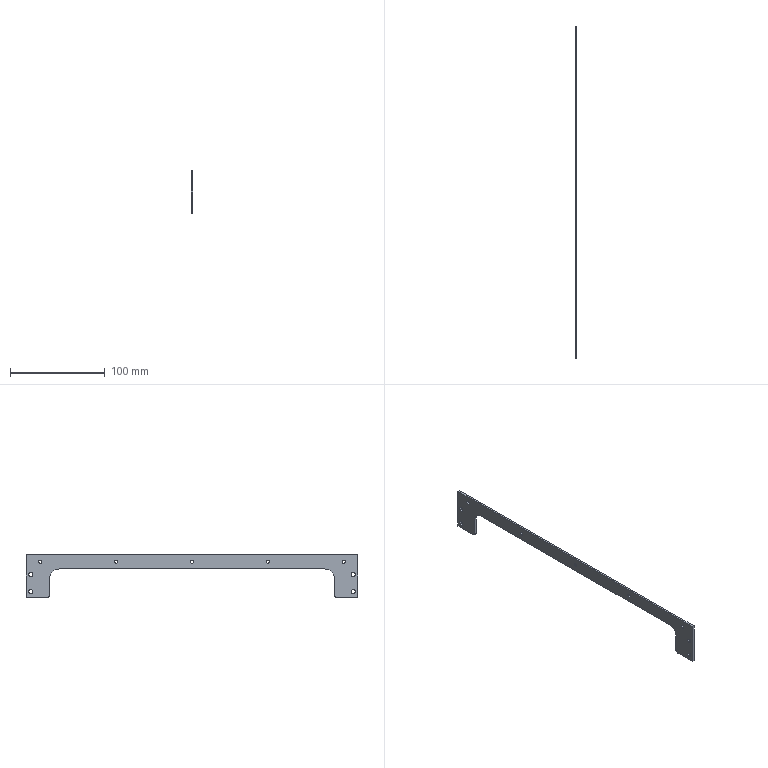Component | SolidWorks | AUTO-SpinDryWashing-01-03000009-1 | 1 solid | 32 faces | box 2 x 350 x 45 mm | volume 13360 mm3 | cylinder 22 | plane 10 | commonest cylinder face diameters 3.4 x10 4.5 x8 20 x2 6 x2 | material AISI 304
build123d program:
from build123d import *

# Parameters (mm, degrees)
SKETCH1_W                = 45
SKETCH1_H                = 350
BOSS_EXTRUDE1_DEPTH      = 1
M3_CLEARANCE_HOLE1_D     = 3.4
M3_CLEARANCE_HOLE1_DEPTH = 10
M3_CLEARANCE_HOLE1_TIP   = 1.021
M4_CLEARANCE_HOLE1_D     = 4.5
M4_CLEARANCE_HOLE1_DEPTH = 10
M4_CLEARANCE_HOLE1_TIP   = 1.352
SKETCH7_W                = 79.155
SKETCH7_H                = 300
CUT_EXTRUDE1_DEPTH       = 10
FILLET1_R                = 10
FILLET2_R                = 3


with BuildPart() as part:
    # Sketch1 → Boss-Extrude1 (new, symmetric)
    with BuildSketch(Plane.XY):
        Rectangle(SKETCH1_W, SKETCH1_H)
    extrude(amount=BOSS_EXTRUDE1_DEPTH, both=True)

    # M3 Clearance Hole1
    with Locations(Plane.XY.offset(1)):
        with Locations((-15, 160), (-15, 80), (-15, 0), (-15, -80), (-15, -160)):
            Hole(M3_CLEARANCE_HOLE1_D / 2, depth=M3_CLEARANCE_HOLE1_DEPTH)
            with Locations((0, 0, -(M3_CLEARANCE_HOLE1_DEPTH + M3_CLEARANCE_HOLE1_TIP / 2))):  # 118° drill point
                Cone(0, M3_CLEARANCE_HOLE1_D / 2, M3_CLEARANCE_HOLE1_TIP, mode=Mode.SUBTRACT)

    # M4 Clearance Hole1
    with Locations(Plane.XY.offset(1)):
        with Locations((-1.5, 170), (16.5, 170), (-1.5, -170), (16.5, -170)):
            Hole(M4_CLEARANCE_HOLE1_D / 2, depth=M4_CLEARANCE_HOLE1_DEPTH)
            with Locations((0, 0, -(M4_CLEARANCE_HOLE1_DEPTH + M4_CLEARANCE_HOLE1_TIP / 2))):  # 118° drill point
                Cone(0, M4_CLEARANCE_HOLE1_D / 2, M4_CLEARANCE_HOLE1_TIP, mode=Mode.SUBTRACT)

    # Sketch7 → Cut-Extrude1 (cut)
    with BuildSketch(Plane.XY.offset(1)):
        with Locations((32.077, 0)):
            Rectangle(SKETCH7_W, SKETCH7_H)
    extrude(amount=-CUT_EXTRUDE1_DEPTH, mode=Mode.SUBTRACT)

    # Fillet1
    fillet1_edges = [part.edges().sort_by_distance(p)[0] for p in [
        (-7.5, -150, 0),
        (-7.5, 150, 0),
    ]]
    fillet(fillet1_edges, radius=FILLET1_R)

    # Fillet2
    fillet2_edges = [part.edges().sort_by_distance(p)[0] for p in [
        (22.5, 150, 0),
        (22.5, -150, 0),
    ]]
    fillet(fillet2_edges, radius=FILLET2_R)


solid = part.part

# Placed as in the assembly
solid = solid.moved(Location((366, 643, 42.5), (0, 90, 0)))
STEP:
#1=CARTESIAN_POINT('',(14.37,32.008,1.821));
#2=VERTEX_POINT('',#1);
#3=CARTESIAN_POINT('',(14.37,32.008,1.644));
#4=VERTEX_POINT('',#3);
#5=CARTESIAN_POINT('',(14.37,32.008,1.732));
#6=DIRECTION('',(1.,-0.,0.));
#7=DIRECTION('',(0.,0.,-1.));
#8=AXIS2_PLACEMENT_3D('',#5,#6,#7);
#9=CIRCLE('',#8,0.08858);
#10=EDGE_CURVE('',#2,#4,#9,.T.);
#11=ORIENTED_EDGE('',*,*,#10,.F.);
#12=CARTESIAN_POINT('',(14.449,32.008,1.821));
#13=VERTEX_POINT('',#12);
#14=CARTESIAN_POINT('',(14.449,32.008,1.821));
#15=DIRECTION('',(1.,-0.,0.));
#16=VECTOR('',#15,39.37);
#17=LINE('',#14,#16);
#18=EDGE_CURVE('',#2,#13,#17,.T.);
#19=ORIENTED_EDGE('',*,*,#18,.T.);
#20=CARTESIAN_POINT('',(14.449,32.008,1.644));
#21=VERTEX_POINT('',#20);
#22=CARTESIAN_POINT('',(14.449,32.008,1.732));
#23=DIRECTION('',(1.,-0.,0.));
#24=DIRECTION('',(0.,0.,-1.));
#25=AXIS2_PLACEMENT_3D('',#22,#23,#24);
#26=CIRCLE('',#25,0.08858);
#27=EDGE_CURVE('',#13,#21,#26,.T.);
#28=ORIENTED_EDGE('',*,*,#27,.T.);
#29=CARTESIAN_POINT('',(14.449,32.008,1.644));
#30=DIRECTION('',(1.,-0.,0.));
#31=VECTOR('',#30,39.37);
#32=LINE('',#29,#31);
#33=EDGE_CURVE('',#4,#21,#32,.T.);
#34=ORIENTED_EDGE('',*,*,#33,.F.);
#35=EDGE_LOOP('',(#11,#19,#28,#34));
#36=FACE_OUTER_BOUND('',#35,.T.);
#37=CARTESIAN_POINT('',(14.449,32.008,1.732));
#38=DIRECTION('',(1.,-0.,0.));
#39=DIRECTION('',(0.,0.,-1.));
#40=AXIS2_PLACEMENT_3D('',#37,#38,#39);
#41=CYLINDRICAL_SURFACE('',#40,0.08858);
#42=ADVANCED_FACE('',(#36),#41,.F.);
#43=CARTESIAN_POINT('',(14.37,32.008,1.112));
#44=VERTEX_POINT('',#43);
#45=CARTESIAN_POINT('',(14.37,32.008,0.935));
#46=VERTEX_POINT('',#45);
#47=CARTESIAN_POINT('',(14.37,32.008,1.024));
#48=DIRECTION('',(1.,-0.,0.));
#49=DIRECTION('',(0.,0.,-1.));
#50=AXIS2_PLACEMENT_3D('',#47,#48,#49);
#51=CIRCLE('',#50,0.08858);
#52=EDGE_CURVE('',#44,#46,#51,.T.);
#53=ORIENTED_EDGE('',*,*,#52,.F.);
#54=CARTESIAN_POINT('',(14.449,32.008,1.112));
#55=VERTEX_POINT('',#54);
#56=CARTESIAN_POINT('',(14.449,32.008,1.112));
#57=DIRECTION('',(1.,-0.,0.));
#58=VECTOR('',#57,39.37);
#59=LINE('',#56,#58);
#60=EDGE_CURVE('',#44,#55,#59,.T.);
#61=ORIENTED_EDGE('',*,*,#60,.T.);
#62=CARTESIAN_POINT('',(14.449,32.008,0.935));
#63=VERTEX_POINT('',#62);
#64=CARTESIAN_POINT('',(14.449,32.008,1.024));
#65=DIRECTION('',(1.,-0.,0.));
#66=DIRECTION('',(0.,0.,-1.));
#67=AXIS2_PLACEMENT_3D('',#64,#65,#66);
#68=CIRCLE('',#67,0.08858);
#69=EDGE_CURVE('',#55,#63,#68,.T.);
#70=ORIENTED_EDGE('',*,*,#69,.T.);
#71=CARTESIAN_POINT('',(14.449,32.008,0.935));
#72=DIRECTION('',(1.,-0.,0.));
#73=VECTOR('',#72,39.37);
#74=LINE('',#71,#73);
#75=EDGE_CURVE('',#46,#63,#74,.T.);
#76=ORIENTED_EDGE('',*,*,#75,.F.);
#77=EDGE_LOOP('',(#53,#61,#70,#76));
#78=FACE_OUTER_BOUND('',#77,.T.);
#79=CARTESIAN_POINT('',(14.449,32.008,1.024));
#80=DIRECTION('',(1.,-0.,0.));
#81=DIRECTION('',(0.,0.,-1.));
#82=AXIS2_PLACEMENT_3D('',#79,#80,#81);
#83=CYLINDRICAL_SURFACE('',#82,0.08858);
#84=ADVANCED_FACE('',(#78),#83,.F.);
#85=CARTESIAN_POINT('',(14.37,18.622,1.821));
#86=VERTEX_POINT('',#85);
#87=CARTESIAN_POINT('',(14.37,18.622,1.644));
#88=VERTEX_POINT('',#87);
#89=CARTESIAN_POINT('',(14.37,18.622,1.732));
#90=DIRECTION('',(1.,-0.,0.));
#91=DIRECTION('',(0.,0.,-1.));
#92=AXIS2_PLACEMENT_3D('',#89,#90,#91);
#93=CIRCLE('',#92,0.08858);
#94=EDGE_CURVE('',#86,#88,#93,.T.);
#95=ORIENTED_EDGE('',*,*,#94,.F.);
#96=CARTESIAN_POINT('',(14.449,18.622,1.821));
#97=VERTEX_POINT('',#96);
#98=CARTESIAN_POINT('',(14.449,18.622,1.821));
#99=DIRECTION('',(1.,-0.,0.));
#100=VECTOR('',#99,39.37);
#101=LINE('',#98,#100);
#102=EDGE_CURVE('',#86,#97,#101,.T.);
#103=ORIENTED_EDGE('',*,*,#102,.T.);
#104=CARTESIAN_POINT('',(14.449,18.622,1.644));
#105=VERTEX_POINT('',#104);
#106=CARTESIAN_POINT('',(14.449,18.622,1.732));
#107=DIRECTION('',(1.,-0.,0.));
#108=DIRECTION('',(0.,0.,-1.));
#109=AXIS2_PLACEMENT_3D('',#106,#107,#108);
#110=CIRCLE('',#109,0.08858);
#111=EDGE_CURVE('',#97,#105,#110,.T.);
#112=ORIENTED_EDGE('',*,*,#111,.T.);
#113=CARTESIAN_POINT('',(14.449,18.622,1.644));
#114=DIRECTION('',(1.,-0.,0.));
#115=VECTOR('',#114,39.37);
#116=LINE('',#113,#115);
#117=EDGE_CURVE('',#88,#105,#116,.T.);
#118=ORIENTED_EDGE('',*,*,#117,.F.);
#119=EDGE_LOOP('',(#95,#103,#112,#118));
#120=FACE_OUTER_BOUND('',#119,.T.);
#121=CARTESIAN_POINT('',(14.449,18.622,1.732));
#122=DIRECTION('',(1.,-0.,0.));
#123=DIRECTION('',(0.,0.,-1.));
#124=AXIS2_PLACEMENT_3D('',#121,#122,#123);
#125=CYLINDRICAL_SURFACE('',#124,0.08858);
#126=ADVANCED_FACE('',(#120),#125,.F.);
#127=CARTESIAN_POINT('',(14.37,18.622,1.112));
#128=VERTEX_POINT('',#127);
#129=CARTESIAN_POINT('',(14.37,18.622,0.935));
#130=VERTEX_POINT('',#129);
#131=CARTESIAN_POINT('',(14.37,18.622,1.024));
#132=DIRECTION('',(1.,-0.,0.));
#133=DIRECTION('',(0.,0.,-1.));
#134=AXIS2_PLACEMENT_3D('',#131,#132,#133);
#135=CIRCLE('',#134,0.08858);
#136=EDGE_CURVE('',#128,#130,#135,.T.);
#137=ORIENTED_EDGE('',*,*,#136,.F.);
#138=CARTESIAN_POINT('',(14.449,18.622,1.112));
#139=VERTEX_POINT('',#138);
#140=CARTESIAN_POINT('',(14.449,18.622,1.112));
#141=DIRECTION('',(1.,-0.,0.));
#142=VECTOR('',#141,39.37);
#143=LINE('',#140,#142);
#144=EDGE_CURVE('',#128,#139,#143,.T.);
#145=ORIENTED_EDGE('',*,*,#144,.T.);
#146=CARTESIAN_POINT('',(14.449,18.622,0.935));
#147=VERTEX_POINT('',#146);
#148=CARTESIAN_POINT('',(14.449,18.622,1.024));
#149=DIRECTION('',(1.,-0.,0.));
#150=DIRECTION('',(0.,0.,-1.));
#151=AXIS2_PLACEMENT_3D('',#148,#149,#150);
#152=CIRCLE('',#151,0.08858);
#153=EDGE_CURVE('',#139,#147,#152,.T.);
#154=ORIENTED_EDGE('',*,*,#153,.T.);
#155=CARTESIAN_POINT('',(14.449,18.622,0.935));
#156=DIRECTION('',(1.,-0.,0.));
#157=VECTOR('',#156,39.37);
#158=LINE('',#155,#157);
#159=EDGE_CURVE('',#130,#147,#158,.T.);
#160=ORIENTED_EDGE('',*,*,#159,.F.);
#161=EDGE_LOOP('',(#137,#145,#154,#160));
#162=FACE_OUTER_BOUND('',#161,.T.);
#163=CARTESIAN_POINT('',(14.449,18.622,1.024));
#164=DIRECTION('',(1.,-0.,0.));
#165=DIRECTION('',(0.,0.,-1.));
#166=AXIS2_PLACEMENT_3D('',#163,#164,#165);
#167=CYLINDRICAL_SURFACE('',#166,0.08858);
#168=ADVANCED_FACE('',(#162),#167,.F.);
#169=CARTESIAN_POINT('',(14.37,31.614,2.331));
#170=VERTEX_POINT('',#169);
#171=CARTESIAN_POINT('',(14.37,31.614,2.197));
#172=VERTEX_POINT('',#171);
#173=CARTESIAN_POINT('',(14.37,31.614,2.264));
#174=DIRECTION('',(1.,-0.,0.));
#175=DIRECTION('',(0.,0.,-1.));
#176=AXIS2_PLACEMENT_3D('',#173,#174,#175);
#177=CIRCLE('',#176,0.06693);
#178=EDGE_CURVE('',#170,#172,#177,.T.);
#179=ORIENTED_EDGE('',*,*,#178,.F.);
#180=CARTESIAN_POINT('',(14.449,31.614,2.331));
#181=VERTEX_POINT('',#180);
#182=CARTESIAN_POINT('',(14.449,31.614,2.331));
#183=DIRECTION('',(1.,-0.,0.));
#184=VECTOR('',#183,39.37);
#185=LINE('',#182,#184);
#186=EDGE_CURVE('',#170,#181,#185,.T.);
#187=ORIENTED_EDGE('',*,*,#186,.T.);
#188=CARTESIAN_POINT('',(14.449,31.614,2.197));
#189=VERTEX_POINT('',#188);
#190=CARTESIAN_POINT('',(14.449,31.614,2.264));
#191=DIRECTION('',(1.,-0.,0.));
#192=DIRECTION('',(0.,0.,-1.));
#193=AXIS2_PLACEMENT_3D('',#190,#191,#192);
#194=CIRCLE('',#193,0.06693);
#195=EDGE_CURVE('',#181,#189,#194,.T.);
#196=ORIENTED_EDGE('',*,*,#195,.T.);
#197=CARTESIAN_POINT('',(14.449,31.614,2.197));
#198=DIRECTION('',(1.,-0.,0.));
#199=VECTOR('',#198,39.37);
#200=LINE('',#197,#199);
#201=EDGE_CURVE('',#172,#189,#200,.T.);
#202=ORIENTED_EDGE('',*,*,#201,.F.);
#203=EDGE_LOOP('',(#179,#187,#196,#202));
#204=FACE_OUTER_BOUND('',#203,.T.);
#205=CARTESIAN_POINT('',(14.449,31.614,2.264));
#206=DIRECTION('',(1.,-0.,0.));
#207=DIRECTION('',(0.,0.,-1.));
#208=AXIS2_PLACEMENT_3D('',#205,#206,#207);
#209=CYLINDRICAL_SURFACE('',#208,0.06693);
#210=ADVANCED_FACE('',(#204),#209,.F.);
#211=CARTESIAN_POINT('',(14.37,28.465,2.331));
#212=VERTEX_POINT('',#211);
#213=CARTESIAN_POINT('',(14.37,28.465,2.197));
#214=VERTEX_POINT('',#213);
#215=CARTESIAN_POINT('',(14.37,28.465,2.264));
#216=DIRECTION('',(1.,-0.,0.));
#217=DIRECTION('',(0.,0.,-1.));
#218=AXIS2_PLACEMENT_3D('',#215,#216,#217);
#219=CIRCLE('',#218,0.06693);
#220=EDGE_CURVE('',#212,#214,#219,.T.);
#221=ORIENTED_EDGE('',*,*,#220,.F.);
#222=CARTESIAN_POINT('',(14.449,28.465,2.331));
#223=VERTEX_POINT('',#222);
#224=CARTESIAN_POINT('',(14.449,28.465,2.331));
#225=DIRECTION('',(1.,-0.,0.));
#226=VECTOR('',#225,39.37);
#227=LINE('',#224,#226);
#228=EDGE_CURVE('',#212,#223,#227,.T.);
#229=ORIENTED_EDGE('',*,*,#228,.T.);
#230=CARTESIAN_POINT('',(14.449,28.465,2.197));
#231=VERTEX_POINT('',#230);
#232=CARTESIAN_POINT('',(14.449,28.465,2.264));
#233=DIRECTION('',(1.,-0.,0.));
#234=DIRECTION('',(0.,0.,-1.));
#235=AXIS2_PLACEMENT_3D('',#232,#233,#234);
#236=CIRCLE('',#235,0.06693);
#237=EDGE_CURVE('',#223,#231,#236,.T.);
#238=ORIENTED_EDGE('',*,*,#237,.T.);
#239=CARTESIAN_POINT('',(14.449,28.465,2.197));
#240=DIRECTION('',(1.,-0.,0.));
#241=VECTOR('',#240,39.37);
#242=LINE('',#239,#241);
#243=EDGE_CURVE('',#214,#231,#242,.T.);
#244=ORIENTED_EDGE('',*,*,#243,.F.);
#245=EDGE_LOOP('',(#221,#229,#238,#244));
#246=FACE_OUTER_BOUND('',#245,.T.);
#247=CARTESIAN_POINT('',(14.449,28.465,2.264));
#248=DIRECTION('',(1.,-0.,0.));
#249=DIRECTION('',(0.,0.,-1.));
#250=AXIS2_PLACEMENT_3D('',#247,#248,#249);
#251=CYLINDRICAL_SURFACE('',#250,0.06693);
#252=ADVANCED_FACE('',(#246),#251,.F.);
#253=CARTESIAN_POINT('',(14.37,25.315,2.331));
#254=VERTEX_POINT('',#253);
#255=CARTESIAN_POINT('',(14.37,25.315,2.197));
#256=VERTEX_POINT('',#255);
#257=CARTESIAN_POINT('',(14.37,25.315,2.264));
#258=DIRECTION('',(1.,-0.,0.));
#259=DIRECTION('',(0.,0.,-1.));
#260=AXIS2_PLACEMENT_3D('',#257,#258,#259);
#261=CIRCLE('',#260,0.06693);
#262=EDGE_CURVE('',#254,#256,#261,.T.);
#263=ORIENTED_EDGE('',*,*,#262,.F.);
#264=CARTESIAN_POINT('',(14.449,25.315,2.331));
#265=VERTEX_POINT('',#264);
#266=CARTESIAN_POINT('',(14.449,25.315,2.331));
#267=DIRECTION('',(1.,-0.,0.));
#268=VECTOR('',#267,39.37);
#269=LINE('',#266,#268);
#270=EDGE_CURVE('',#254,#265,#269,.T.);
#271=ORIENTED_EDGE('',*,*,#270,.T.);
#272=CARTESIAN_POINT('',(14.449,25.315,2.197));
#273=VERTEX_POINT('',#272);
#274=CARTESIAN_POINT('',(14.449,25.315,2.264));
#275=DIRECTION('',(1.,-0.,0.));
#276=DIRECTION('',(0.,0.,-1.));
#277=AXIS2_PLACEMENT_3D('',#274,#275,#276);
#278=CIRCLE('',#277,0.06693);
#279=EDGE_CURVE('',#265,#273,#278,.T.);
#280=ORIENTED_EDGE('',*,*,#279,.T.);
#281=CARTESIAN_POINT('',(14.449,25.315,2.197));
#282=DIRECTION('',(1.,-0.,0.));
#283=VECTOR('',#282,39.37);
#284=LINE('',#281,#283);
#285=EDGE_CURVE('',#256,#273,#284,.T.);
#286=ORIENTED_EDGE('',*,*,#285,.F.);
#287=EDGE_LOOP('',(#263,#271,#280,#286));
#288=FACE_OUTER_BOUND('',#287,.T.);
#289=CARTESIAN_POINT('',(14.449,25.315,2.264));
#290=DIRECTION('',(1.,-0.,0.));
#291=DIRECTION('',(0.,0.,-1.));
#292=AXIS2_PLACEMENT_3D('',#289,#290,#291);
#293=CYLINDRICAL_SURFACE('',#292,0.06693);
#294=ADVANCED_FACE('',(#288),#293,.F.);
#295=CARTESIAN_POINT('',(14.37,22.165,2.331));
#296=VERTEX_POINT('',#295);
#297=CARTESIAN_POINT('',(14.37,22.165,2.197));
#298=VERTEX_POINT('',#297);
#299=CARTESIAN_POINT('',(14.37,22.165,2.264));
#300=DIRECTION('',(1.,-0.,0.));
#301=DIRECTION('',(0.,0.,-1.));
#302=AXIS2_PLACEMENT_3D('',#299,#300,#301);
#303=CIRCLE('',#302,0.06693);
#304=EDGE_CURVE('',#296,#298,#303,.T.);
#305=ORIENTED_EDGE('',*,*,#304,.F.);
#306=CARTESIAN_POINT('',(14.449,22.165,2.331));
#307=VERTEX_POINT('',#306);
#308=CARTESIAN_POINT('',(14.449,22.165,2.331));
#309=DIRECTION('',(1.,-0.,0.));
#310=VECTOR('',#309,39.37);
#311=LINE('',#308,#310);
#312=EDGE_CURVE('',#296,#307,#311,.T.);
#313=ORIENTED_EDGE('',*,*,#312,.T.);
#314=CARTESIAN_POINT('',(14.449,22.165,2.197));
#315=VERTEX_POINT('',#314);
#316=CARTESIAN_POINT('',(14.449,22.165,2.264));
#317=DIRECTION('',(1.,-0.,0.));
#318=DIRECTION('',(0.,0.,-1.));
#319=AXIS2_PLACEMENT_3D('',#316,#317,#318);
#320=CIRCLE('',#319,0.06693);
#321=EDGE_CURVE('',#307,#315,#320,.T.);
#322=ORIENTED_EDGE('',*,*,#321,.T.);
#323=CARTESIAN_POINT('',(14.449,22.165,2.197));
#324=DIRECTION('',(1.,-0.,0.));
#325=VECTOR('',#324,39.37);
#326=LINE('',#323,#325);
#327=EDGE_CURVE('',#298,#315,#326,.T.);
#328=ORIENTED_EDGE('',*,*,#327,.F.);
#329=EDGE_LOOP('',(#305,#313,#322,#328));
#330=FACE_OUTER_BOUND('',#329,.T.);
#331=CARTESIAN_POINT('',(14.449,22.165,2.264));
#332=DIRECTION('',(1.,-0.,0.));
#333=DIRECTION('',(0.,0.,-1.));
#334=AXIS2_PLACEMENT_3D('',#331,#332,#333);
#335=CYLINDRICAL_SURFACE('',#334,0.06693);
#336=ADVANCED_FACE('',(#330),#335,.F.);
#337=CARTESIAN_POINT('',(14.37,19.016,2.331));
#338=VERTEX_POINT('',#337);
#339=CARTESIAN_POINT('',(14.37,19.016,2.197));
#340=VERTEX_POINT('',#339);
#341=CARTESIAN_POINT('',(14.37,19.016,2.264));
#342=DIRECTION('',(1.,-0.,0.));
#343=DIRECTION('',(0.,0.,-1.));
#344=AXIS2_PLACEMENT_3D('',#341,#342,#343);
#345=CIRCLE('',#344,0.06693);
#346=EDGE_CURVE('',#338,#340,#345,.T.);
#347=ORIENTED_EDGE('',*,*,#346,.F.);
#348=CARTESIAN_POINT('',(14.449,19.016,2.331));
#349=VERTEX_POINT('',#348);
#350=CARTESIAN_POINT('',(14.449,19.016,2.331));
#351=DIRECTION('',(1.,-0.,0.));
#352=VECTOR('',#351,39.37);
#353=LINE('',#350,#352);
#354=EDGE_CURVE('',#338,#349,#353,.T.);
#355=ORIENTED_EDGE('',*,*,#354,.T.);
#356=CARTESIAN_POINT('',(14.449,19.016,2.197));
#357=VERTEX_POINT('',#356);
#358=CARTESIAN_POINT('',(14.449,19.016,2.264));
#359=DIRECTION('',(1.,-0.,0.));
#360=DIRECTION('',(0.,0.,-1.));
#361=AXIS2_PLACEMENT_3D('',#358,#359,#360);
#362=CIRCLE('',#361,0.06693);
#363=EDGE_CURVE('',#349,#357,#362,.T.);
#364=ORIENTED_EDGE('',*,*,#363,.T.);
#365=CARTESIAN_POINT('',(14.449,19.016,2.197));
#366=DIRECTION('',(1.,-0.,0.));
#367=VECTOR('',#366,39.37);
#368=LINE('',#365,#367);
#369=EDGE_CURVE('',#340,#357,#368,.T.);
#370=ORIENTED_EDGE('',*,*,#369,.F.);
#371=EDGE_LOOP('',(#347,#355,#364,#370));
#372=FACE_OUTER_BOUND('',#371,.T.);
#373=CARTESIAN_POINT('',(14.449,19.016,2.264));
#374=DIRECTION('',(1.,-0.,0.));
#375=DIRECTION('',(0.,0.,-1.));
#376=AXIS2_PLACEMENT_3D('',#373,#374,#375);
#377=CYLINDRICAL_SURFACE('',#376,0.06693);
#378=ADVANCED_FACE('',(#372),#377,.F.);
#379=CARTESIAN_POINT('',(14.449,32.205,0.7874));
#380=VERTEX_POINT('',#379);
#381=CARTESIAN_POINT('',(14.449,31.339,0.7874));
#382=VERTEX_POINT('',#381);
#383=CARTESIAN_POINT('',(14.449,25.315,0.7874));
#384=DIRECTION('',(-0.,-1.,-0.));
#385=VECTOR('',#384,39.37);
#386=LINE('',#383,#385);
#387=EDGE_CURVE('',#380,#382,#386,.T.);
#388=ORIENTED_EDGE('',*,*,#387,.T.);
#389=CARTESIAN_POINT('',(14.37,31.339,0.7874));
#390=VERTEX_POINT('',#389);
#391=CARTESIAN_POINT('',(14.37,31.339,0.7874));
#392=DIRECTION('',(-1.,0.,-0.));
#393=VECTOR('',#392,39.37);
#394=LINE('',#391,#393);
#395=EDGE_CURVE('',#382,#390,#394,.T.);
#396=ORIENTED_EDGE('',*,*,#395,.T.);
#397=CARTESIAN_POINT('',(14.37,32.205,0.7874));
#398=VERTEX_POINT('',#397);
#399=CARTESIAN_POINT('',(14.37,25.315,0.7874));
#400=DIRECTION('',(-0.,-1.,-0.));
#401=VECTOR('',#400,39.37);
#402=LINE('',#399,#401);
#403=EDGE_CURVE('',#398,#390,#402,.T.);
#404=ORIENTED_EDGE('',*,*,#403,.F.);
#405=CARTESIAN_POINT('',(14.449,32.205,0.7874));
#406=DIRECTION('',(-1.,0.,-0.));
#407=VECTOR('',#406,39.37);
#408=LINE('',#405,#407);
#409=EDGE_CURVE('',#380,#398,#408,.T.);
#410=ORIENTED_EDGE('',*,*,#409,.F.);
#411=EDGE_LOOP('',(#388,#396,#404,#410));
#412=FACE_OUTER_BOUND('',#411,.T.);
#413=CARTESIAN_POINT('',(14.449,25.315,0.7874));
#414=DIRECTION('',(0.,0.,-1.));
#415=DIRECTION('',(0.,1.,0.));
#416=AXIS2_PLACEMENT_3D('',#413,#414,#415);
#417=PLANE('',#416);
#418=ADVANCED_FACE('',(#412),#417,.T.);
#419=CARTESIAN_POINT('',(14.37,19.291,0.7874));
#420=VERTEX_POINT('',#419);
#421=CARTESIAN_POINT('',(14.37,18.425,0.7874));
#422=VERTEX_POINT('',#421);
#423=CARTESIAN_POINT('',(14.37,25.315,0.7874));
#424=DIRECTION('',(-0.,-1.,-0.));
#425=VECTOR('',#424,39.37);
#426=LINE('',#423,#425);
#427=EDGE_CURVE('',#420,#422,#426,.T.);
#428=ORIENTED_EDGE('',*,*,#427,.F.);
#429=CARTESIAN_POINT('',(14.449,19.291,0.7874));
#430=VERTEX_POINT('',#429);
#431=CARTESIAN_POINT('',(14.449,19.291,0.7874));
#432=DIRECTION('',(1.,-0.,0.));
#433=VECTOR('',#432,39.37);
#434=LINE('',#431,#433);
#435=EDGE_CURVE('',#420,#430,#434,.T.);
#436=ORIENTED_EDGE('',*,*,#435,.T.);
#437=CARTESIAN_POINT('',(14.449,18.425,0.7874));
#438=VERTEX_POINT('',#437);
#439=CARTESIAN_POINT('',(14.449,25.315,0.7874));
#440=DIRECTION('',(-0.,-1.,-0.));
#441=VECTOR('',#440,39.37);
#442=LINE('',#439,#441);
#443=EDGE_CURVE('',#430,#438,#442,.T.);
#444=ORIENTED_EDGE('',*,*,#443,.T.);
#445=CARTESIAN_POINT('',(14.449,18.425,0.7874));
#446=DIRECTION('',(-1.,0.,-0.));
#447=VECTOR('',#446,39.37);
#448=LINE('',#445,#447);
#449=EDGE_CURVE('',#438,#422,#448,.T.);
#450=ORIENTED_EDGE('',*,*,#449,.T.);
#451=EDGE_LOOP('',(#428,#436,#444,#450));
#452=FACE_OUTER_BOUND('',#451,.T.);
#453=CARTESIAN_POINT('',(14.449,25.315,0.7874));
#454=DIRECTION('',(0.,0.,-1.));
#455=DIRECTION('',(0.,1.,0.));
#456=AXIS2_PLACEMENT_3D('',#453,#454,#455);
#457=PLANE('',#456);
#458=ADVANCED_FACE('',(#452),#457,.T.);
#459=CARTESIAN_POINT('',(14.37,32.205,2.559));
#460=VERTEX_POINT('',#459);
#461=CARTESIAN_POINT('',(14.37,32.205,1.673));
#462=DIRECTION('',(0.,-0.,-1.));
#463=VECTOR('',#462,39.37);
#464=LINE('',#461,#463);
#465=EDGE_CURVE('',#460,#398,#464,.T.);
#466=ORIENTED_EDGE('',*,*,#465,.F.);
#467=CARTESIAN_POINT('',(14.449,32.205,2.559));
#468=VERTEX_POINT('',#467);
#469=CARTESIAN_POINT('',(14.449,32.205,2.559));
#470=DIRECTION('',(-1.,0.,-0.));
#471=VECTOR('',#470,39.37);
#472=LINE('',#469,#471);
#473=EDGE_CURVE('',#468,#460,#472,.T.);
#474=ORIENTED_EDGE('',*,*,#473,.F.);
#475=CARTESIAN_POINT('',(14.449,32.205,1.673));
#476=DIRECTION('',(0.,-0.,-1.));
#477=VECTOR('',#476,39.37);
#478=LINE('',#475,#477);
#479=EDGE_CURVE('',#468,#380,#478,.T.);
#480=ORIENTED_EDGE('',*,*,#479,.T.);
#481=ORIENTED_EDGE('',*,*,#409,.T.);
#482=EDGE_LOOP('',(#466,#474,#480,#481));
#483=FACE_OUTER_BOUND('',#482,.T.);
#484=CARTESIAN_POINT('',(14.449,32.205,1.673));
#485=DIRECTION('',(0.,1.,-0.));
#486=DIRECTION('',(1.,-0.,0.));
#487=AXIS2_PLACEMENT_3D('',#484,#485,#486);
#488=PLANE('',#487);
#489=ADVANCED_FACE('',(#483),#488,.T.);
#490=CARTESIAN_POINT('',(14.37,18.425,2.559));
#491=VERTEX_POINT('',#490);
#492=CARTESIAN_POINT('',(14.37,25.315,2.559));
#493=DIRECTION('',(-0.,-1.,-0.));
#494=VECTOR('',#493,39.37);
#495=LINE('',#492,#494);
#496=EDGE_CURVE('',#460,#491,#495,.T.);
#497=ORIENTED_EDGE('',*,*,#496,.T.);
#498=CARTESIAN_POINT('',(14.449,18.425,2.559));
#499=VERTEX_POINT('',#498);
#500=CARTESIAN_POINT('',(14.449,18.425,2.559));
#501=DIRECTION('',(-1.,0.,-0.));
#502=VECTOR('',#501,39.37);
#503=LINE('',#500,#502);
#504=EDGE_CURVE('',#499,#491,#503,.T.);
#505=ORIENTED_EDGE('',*,*,#504,.F.);
#506=CARTESIAN_POINT('',(14.449,25.315,2.559));
#507=DIRECTION('',(-0.,-1.,-0.));
#508=VECTOR('',#507,39.37);
#509=LINE('',#506,#508);
#510=EDGE_CURVE('',#468,#499,#509,.T.);
#511=ORIENTED_EDGE('',*,*,#510,.F.);
#512=ORIENTED_EDGE('',*,*,#473,.T.);
#513=EDGE_LOOP('',(#497,#505,#511,#512));
#514=FACE_OUTER_BOUND('',#513,.T.);
#515=CARTESIAN_POINT('',(14.449,25.315,2.559));
#516=DIRECTION('',(0.,0.,-1.));
#517=DIRECTION('',(0.,1.,0.));
#518=AXIS2_PLACEMENT_3D('',#515,#516,#517);
#519=PLANE('',#518);
#520=ADVANCED_FACE('',(#514),#519,.F.);
#521=CARTESIAN_POINT('',(14.37,18.425,1.673));
#522=DIRECTION('',(0.,-0.,-1.));
#523=VECTOR('',#522,39.37);
#524=LINE('',#521,#523);
#525=EDGE_CURVE('',#491,#422,#524,.T.);
#526=ORIENTED_EDGE('',*,*,#525,.T.);
#527=ORIENTED_EDGE('',*,*,#449,.F.);
#528=CARTESIAN_POINT('',(14.449,18.425,1.673));
#529=DIRECTION('',(0.,-0.,-1.));
#530=VECTOR('',#529,39.37);
#531=LINE('',#528,#530);
#532=EDGE_CURVE('',#499,#438,#531,.T.);
#533=ORIENTED_EDGE('',*,*,#532,.F.);
#534=ORIENTED_EDGE('',*,*,#504,.T.);
#535=EDGE_LOOP('',(#526,#527,#533,#534));
#536=FACE_OUTER_BOUND('',#535,.T.);
#537=CARTESIAN_POINT('',(14.449,18.425,1.673));
#538=DIRECTION('',(0.,1.,-0.));
#539=DIRECTION('',(1.,-0.,0.));
#540=AXIS2_PLACEMENT_3D('',#537,#538,#539);
#541=PLANE('',#540);
#542=ADVANCED_FACE('',(#536),#541,.F.);
#543=ORIENTED_EDGE('',*,*,#443,.F.);
#544=CARTESIAN_POINT('',(14.449,19.409,0.9055));
#545=VERTEX_POINT('',#544);
#546=CARTESIAN_POINT('',(14.449,19.291,0.9055));
#547=DIRECTION('',(1.,-0.,0.));
#548=DIRECTION('',(0.,0.,-1.));
#549=AXIS2_PLACEMENT_3D('',#546,#547,#548);
#550=CIRCLE('',#549,0.1181);
#551=EDGE_CURVE('',#430,#545,#550,.T.);
#552=ORIENTED_EDGE('',*,*,#551,.T.);
#553=CARTESIAN_POINT('',(14.449,19.409,1.575));
#554=VERTEX_POINT('',#553);
#555=CARTESIAN_POINT('',(14.449,19.409,1.969));
#556=DIRECTION('',(0.,-0.,-1.));
#557=VECTOR('',#556,39.37);
#558=LINE('',#555,#557);
#559=EDGE_CURVE('',#554,#545,#558,.T.);
#560=ORIENTED_EDGE('',*,*,#559,.F.);
#561=CARTESIAN_POINT('',(14.449,19.803,1.969));
#562=VERTEX_POINT('',#561);
#563=CARTESIAN_POINT('',(14.449,19.803,1.575));
#564=DIRECTION('',(-1.,0.,-0.));
#565=DIRECTION('',(0.,0.,-1.));
#566=AXIS2_PLACEMENT_3D('',#563,#564,#565);
#567=CIRCLE('',#566,0.3937);
#568=EDGE_CURVE('',#554,#562,#567,.T.);
#569=ORIENTED_EDGE('',*,*,#568,.T.);
#570=CARTESIAN_POINT('',(14.449,30.827,1.969));
#571=VERTEX_POINT('',#570);
#572=CARTESIAN_POINT('',(14.449,31.22,1.969));
#573=DIRECTION('',(-0.,-1.,0.));
#574=VECTOR('',#573,39.37);
#575=LINE('',#572,#574);
#576=EDGE_CURVE('',#571,#562,#575,.T.);
#577=ORIENTED_EDGE('',*,*,#576,.F.);
#578=CARTESIAN_POINT('',(14.449,31.22,1.575));
#579=VERTEX_POINT('',#578);
#580=CARTESIAN_POINT('',(14.449,30.827,1.575));
#581=DIRECTION('',(-1.,0.,-0.));
#582=DIRECTION('',(0.,0.,-1.));
#583=AXIS2_PLACEMENT_3D('',#580,#581,#582);
#584=CIRCLE('',#583,0.3937);
#585=EDGE_CURVE('',#571,#579,#584,.T.);
#586=ORIENTED_EDGE('',*,*,#585,.T.);
#587=CARTESIAN_POINT('',(14.449,31.22,0.9055));
#588=VERTEX_POINT('',#587);
#589=CARTESIAN_POINT('',(14.449,31.22,1.969));
#590=DIRECTION('',(-0.,0.,1.));
#591=VECTOR('',#590,39.37);
#592=LINE('',#589,#591);
#593=EDGE_CURVE('',#588,#579,#592,.T.);
#594=ORIENTED_EDGE('',*,*,#593,.F.);
#595=CARTESIAN_POINT('',(14.449,31.339,0.9055));
#596=DIRECTION('',(1.,-0.,0.));
#597=DIRECTION('',(0.,0.,-1.));
#598=AXIS2_PLACEMENT_3D('',#595,#596,#597);
#599=CIRCLE('',#598,0.1181);
#600=EDGE_CURVE('',#588,#382,#599,.T.);
#601=ORIENTED_EDGE('',*,*,#600,.T.);
#602=ORIENTED_EDGE('',*,*,#387,.F.);
#603=ORIENTED_EDGE('',*,*,#479,.F.);
#604=ORIENTED_EDGE('',*,*,#510,.T.);
#605=ORIENTED_EDGE('',*,*,#532,.T.);
#606=EDGE_LOOP('',(#543,#552,#560,#569,#577,#586,#594,#601,#602,#603,#604,#605));
#607=FACE_OUTER_BOUND('',#606,.T.);
#608=CARTESIAN_POINT('',(14.449,32.008,1.732));
#609=DIRECTION('',(1.,-0.,0.));
#610=DIRECTION('',(0.,0.,-1.));
#611=AXIS2_PLACEMENT_3D('',#608,#609,#610);
#612=CIRCLE('',#611,0.08858);
#613=EDGE_CURVE('',#21,#13,#612,.T.);
#614=ORIENTED_EDGE('',*,*,#613,.F.);
#615=ORIENTED_EDGE('',*,*,#27,.F.);
#616=EDGE_LOOP('',(#614,#615));
#617=FACE_BOUND('',#616,.T.);
#618=CARTESIAN_POINT('',(14.449,32.008,1.024));
#619=DIRECTION('',(1.,-0.,0.));
#620=DIRECTION('',(0.,0.,-1.));
#621=AXIS2_PLACEMENT_3D('',#618,#619,#620);
#622=CIRCLE('',#621,0.08858);
#623=EDGE_CURVE('',#63,#55,#622,.T.);
#624=ORIENTED_EDGE('',*,*,#623,.F.);
#625=ORIENTED_EDGE('',*,*,#69,.F.);
#626=EDGE_LOOP('',(#624,#625));
#627=FACE_BOUND('',#626,.T.);
#628=CARTESIAN_POINT('',(14.449,18.622,1.732));
#629=DIRECTION('',(1.,-0.,0.));
#630=DIRECTION('',(0.,0.,-1.));
#631=AXIS2_PLACEMENT_3D('',#628,#629,#630);
#632=CIRCLE('',#631,0.08858);
#633=EDGE_CURVE('',#105,#97,#632,.T.);
#634=ORIENTED_EDGE('',*,*,#633,.F.);
#635=ORIENTED_EDGE('',*,*,#111,.F.);
#636=EDGE_LOOP('',(#634,#635));
#637=FACE_BOUND('',#636,.T.);
#638=CARTESIAN_POINT('',(14.449,18.622,1.024));
#639=DIRECTION('',(1.,-0.,0.));
#640=DIRECTION('',(0.,0.,-1.));
#641=AXIS2_PLACEMENT_3D('',#638,#639,#640);
#642=CIRCLE('',#641,0.08858);
#643=EDGE_CURVE('',#147,#139,#642,.T.);
#644=ORIENTED_EDGE('',*,*,#643,.F.);
#645=ORIENTED_EDGE('',*,*,#153,.F.);
#646=EDGE_LOOP('',(#644,#645));
#647=FACE_BOUND('',#646,.T.);
#648=CARTESIAN_POINT('',(14.449,31.614,2.264));
#649=DIRECTION('',(1.,-0.,0.));
#650=DIRECTION('',(0.,0.,-1.));
#651=AXIS2_PLACEMENT_3D('',#648,#649,#650);
#652=CIRCLE('',#651,0.06693);
#653=EDGE_CURVE('',#189,#181,#652,.T.);
#654=ORIENTED_EDGE('',*,*,#653,.F.);
#655=ORIENTED_EDGE('',*,*,#195,.F.);
#656=EDGE_LOOP('',(#654,#655));
#657=FACE_BOUND('',#656,.T.);
#658=CARTESIAN_POINT('',(14.449,28.465,2.264));
#659=DIRECTION('',(1.,-0.,0.));
#660=DIRECTION('',(0.,0.,-1.));
#661=AXIS2_PLACEMENT_3D('',#658,#659,#660);
#662=CIRCLE('',#661,0.06693);
#663=EDGE_CURVE('',#231,#223,#662,.T.);
#664=ORIENTED_EDGE('',*,*,#663,.F.);
#665=ORIENTED_EDGE('',*,*,#237,.F.);
#666=EDGE_LOOP('',(#664,#665));
#667=FACE_BOUND('',#666,.T.);
#668=CARTESIAN_POINT('',(14.449,25.315,2.264));
#669=DIRECTION('',(1.,-0.,0.));
#670=DIRECTION('',(0.,0.,-1.));
#671=AXIS2_PLACEMENT_3D('',#668,#669,#670);
#672=CIRCLE('',#671,0.06693);
#673=EDGE_CURVE('',#273,#265,#672,.T.);
#674=ORIENTED_EDGE('',*,*,#673,.F.);
#675=ORIENTED_EDGE('',*,*,#279,.F.);
#676=EDGE_LOOP('',(#674,#675));
#677=FACE_BOUND('',#676,.T.);
#678=CARTESIAN_POINT('',(14.449,22.165,2.264));
#679=DIRECTION('',(1.,-0.,0.));
#680=DIRECTION('',(0.,0.,-1.));
#681=AXIS2_PLACEMENT_3D('',#678,#679,#680);
#682=CIRCLE('',#681,0.06693);
#683=EDGE_CURVE('',#315,#307,#682,.T.);
#684=ORIENTED_EDGE('',*,*,#683,.F.);
#685=ORIENTED_EDGE('',*,*,#321,.F.);
#686=EDGE_LOOP('',(#684,#685));
#687=FACE_BOUND('',#686,.T.);
#688=CARTESIAN_POINT('',(14.449,19.016,2.264));
#689=DIRECTION('',(1.,-0.,0.));
#690=DIRECTION('',(0.,0.,-1.));
#691=AXIS2_PLACEMENT_3D('',#688,#689,#690);
#692=CIRCLE('',#691,0.06693);
#693=EDGE_CURVE('',#357,#349,#692,.T.);
#694=ORIENTED_EDGE('',*,*,#693,.F.);
#695=ORIENTED_EDGE('',*,*,#363,.F.);
#696=EDGE_LOOP('',(#694,#695));
#697=FACE_BOUND('',#696,.T.);
#698=CARTESIAN_POINT('',(14.449,25.315,1.673));
#699=DIRECTION('',(1.,-0.,0.));
#700=DIRECTION('',(0.,-0.,-1.));
#701=AXIS2_PLACEMENT_3D('',#698,#699,#700);
#702=PLANE('',#701);
#703=ADVANCED_FACE('',(#607,#617,#627,#637,#647,#657,#667,#677,#687,#697),#702,.T.);
#704=CARTESIAN_POINT('',(14.37,32.008,1.732));
#705=DIRECTION('',(1.,-0.,0.));
#706=DIRECTION('',(0.,0.,-1.));
#707=AXIS2_PLACEMENT_3D('',#704,#705,#706);
#708=CIRCLE('',#707,0.08858);
#709=EDGE_CURVE('',#4,#2,#708,.T.);
#710=ORIENTED_EDGE('',*,*,#709,.T.);
#711=ORIENTED_EDGE('',*,*,#10,.T.);
#712=EDGE_LOOP('',(#710,#711));
#713=FACE_BOUND('',#712,.T.);
#714=CARTESIAN_POINT('',(14.37,32.008,1.024));
#715=DIRECTION('',(1.,-0.,0.));
#716=DIRECTION('',(0.,0.,-1.));
#717=AXIS2_PLACEMENT_3D('',#714,#715,#716);
#718=CIRCLE('',#717,0.08858);
#719=EDGE_CURVE('',#46,#44,#718,.T.);
#720=ORIENTED_EDGE('',*,*,#719,.T.);
#721=ORIENTED_EDGE('',*,*,#52,.T.);
#722=EDGE_LOOP('',(#720,#721));
#723=FACE_BOUND('',#722,.T.);
#724=CARTESIAN_POINT('',(14.37,18.622,1.732));
#725=DIRECTION('',(1.,-0.,0.));
#726=DIRECTION('',(0.,0.,-1.));
#727=AXIS2_PLACEMENT_3D('',#724,#725,#726);
#728=CIRCLE('',#727,0.08858);
#729=EDGE_CURVE('',#88,#86,#728,.T.);
#730=ORIENTED_EDGE('',*,*,#729,.T.);
#731=ORIENTED_EDGE('',*,*,#94,.T.);
#732=EDGE_LOOP('',(#730,#731));
#733=FACE_BOUND('',#732,.T.);
#734=CARTESIAN_POINT('',(14.37,18.622,1.024));
#735=DIRECTION('',(1.,-0.,0.));
#736=DIRECTION('',(0.,0.,-1.));
#737=AXIS2_PLACEMENT_3D('',#734,#735,#736);
#738=CIRCLE('',#737,0.08858);
#739=EDGE_CURVE('',#130,#128,#738,.T.);
#740=ORIENTED_EDGE('',*,*,#739,.T.);
#741=ORIENTED_EDGE('',*,*,#136,.T.);
#742=EDGE_LOOP('',(#740,#741));
#743=FACE_BOUND('',#742,.T.);
#744=CARTESIAN_POINT('',(14.37,31.614,2.264));
#745=DIRECTION('',(1.,-0.,0.));
#746=DIRECTION('',(0.,0.,-1.));
#747=AXIS2_PLACEMENT_3D('',#744,#745,#746);
#748=CIRCLE('',#747,0.06693);
#749=EDGE_CURVE('',#172,#170,#748,.T.);
#750=ORIENTED_EDGE('',*,*,#749,.T.);
#751=ORIENTED_EDGE('',*,*,#178,.T.);
#752=EDGE_LOOP('',(#750,#751));
#753=FACE_BOUND('',#752,.T.);
#754=CARTESIAN_POINT('',(14.37,28.465,2.264));
#755=DIRECTION('',(1.,-0.,0.));
#756=DIRECTION('',(0.,0.,-1.));
#757=AXIS2_PLACEMENT_3D('',#754,#755,#756);
#758=CIRCLE('',#757,0.06693);
#759=EDGE_CURVE('',#214,#212,#758,.T.);
#760=ORIENTED_EDGE('',*,*,#759,.T.);
#761=ORIENTED_EDGE('',*,*,#220,.T.);
#762=EDGE_LOOP('',(#760,#761));
#763=FACE_BOUND('',#762,.T.);
#764=CARTESIAN_POINT('',(14.37,25.315,2.264));
#765=DIRECTION('',(1.,-0.,0.));
#766=DIRECTION('',(0.,0.,-1.));
#767=AXIS2_PLACEMENT_3D('',#764,#765,#766);
#768=CIRCLE('',#767,0.06693);
#769=EDGE_CURVE('',#256,#254,#768,.T.);
#770=ORIENTED_EDGE('',*,*,#769,.T.);
#771=ORIENTED_EDGE('',*,*,#262,.T.);
#772=EDGE_LOOP('',(#770,#771));
#773=FACE_BOUND('',#772,.T.);
#774=CARTESIAN_POINT('',(14.37,22.165,2.264));
#775=DIRECTION('',(1.,-0.,0.));
#776=DIRECTION('',(0.,0.,-1.));
#777=AXIS2_PLACEMENT_3D('',#774,#775,#776);
#778=CIRCLE('',#777,0.06693);
#779=EDGE_CURVE('',#298,#296,#778,.T.);
#780=ORIENTED_EDGE('',*,*,#779,.T.);
#781=ORIENTED_EDGE('',*,*,#304,.T.);
#782=EDGE_LOOP('',(#780,#781));
#783=FACE_BOUND('',#782,.T.);
#784=CARTESIAN_POINT('',(14.37,19.016,2.264));
#785=DIRECTION('',(1.,-0.,0.));
#786=DIRECTION('',(0.,0.,-1.));
#787=AXIS2_PLACEMENT_3D('',#784,#785,#786);
#788=CIRCLE('',#787,0.06693);
#789=EDGE_CURVE('',#340,#338,#788,.T.);
#790=ORIENTED_EDGE('',*,*,#789,.T.);
#791=ORIENTED_EDGE('',*,*,#346,.T.);
#792=EDGE_LOOP('',(#790,#791));
#793=FACE_BOUND('',#792,.T.);
#794=CARTESIAN_POINT('',(14.37,19.409,1.575));
#795=VERTEX_POINT('',#794);
#796=CARTESIAN_POINT('',(14.37,19.409,0.9055));
#797=VERTEX_POINT('',#796);
#798=CARTESIAN_POINT('',(14.37,19.409,1.673));
#799=DIRECTION('',(0.,-0.,-1.));
#800=VECTOR('',#799,39.37);
#801=LINE('',#798,#800);
#802=EDGE_CURVE('',#795,#797,#801,.T.);
#803=ORIENTED_EDGE('',*,*,#802,.T.);
#804=CARTESIAN_POINT('',(14.37,19.291,0.9055));
#805=DIRECTION('',(-1.,0.,-0.));
#806=DIRECTION('',(0.,0.,-1.));
#807=AXIS2_PLACEMENT_3D('',#804,#805,#806);
#808=CIRCLE('',#807,0.1181);
#809=EDGE_CURVE('',#797,#420,#808,.T.);
#810=ORIENTED_EDGE('',*,*,#809,.T.);
#811=ORIENTED_EDGE('',*,*,#427,.T.);
#812=ORIENTED_EDGE('',*,*,#525,.F.);
#813=ORIENTED_EDGE('',*,*,#496,.F.);
#814=ORIENTED_EDGE('',*,*,#465,.T.);
#815=ORIENTED_EDGE('',*,*,#403,.T.);
#816=CARTESIAN_POINT('',(14.37,31.22,0.9055));
#817=VERTEX_POINT('',#816);
#818=CARTESIAN_POINT('',(14.37,31.339,0.9055));
#819=DIRECTION('',(-1.,0.,-0.));
#820=DIRECTION('',(0.,0.,-1.));
#821=AXIS2_PLACEMENT_3D('',#818,#819,#820);
#822=CIRCLE('',#821,0.1181);
#823=EDGE_CURVE('',#390,#817,#822,.T.);
#824=ORIENTED_EDGE('',*,*,#823,.T.);
#825=CARTESIAN_POINT('',(14.37,31.22,1.575));
#826=VERTEX_POINT('',#825);
#827=CARTESIAN_POINT('',(14.37,31.22,1.673));
#828=DIRECTION('',(-0.,0.,1.));
#829=VECTOR('',#828,39.37);
#830=LINE('',#827,#829);
#831=EDGE_CURVE('',#817,#826,#830,.T.);
#832=ORIENTED_EDGE('',*,*,#831,.T.);
#833=CARTESIAN_POINT('',(14.37,30.827,1.969));
#834=VERTEX_POINT('',#833);
#835=CARTESIAN_POINT('',(14.37,30.827,1.575));
#836=DIRECTION('',(1.,-0.,0.));
#837=DIRECTION('',(0.,0.,-1.));
#838=AXIS2_PLACEMENT_3D('',#835,#836,#837);
#839=CIRCLE('',#838,0.3937);
#840=EDGE_CURVE('',#826,#834,#839,.T.);
#841=ORIENTED_EDGE('',*,*,#840,.T.);
#842=CARTESIAN_POINT('',(14.37,19.803,1.969));
#843=VERTEX_POINT('',#842);
#844=CARTESIAN_POINT('',(14.37,25.315,1.969));
#845=DIRECTION('',(-0.,-1.,0.));
#846=VECTOR('',#845,39.37);
#847=LINE('',#844,#846);
#848=EDGE_CURVE('',#834,#843,#847,.T.);
#849=ORIENTED_EDGE('',*,*,#848,.T.);
#850=CARTESIAN_POINT('',(14.37,19.803,1.575));
#851=DIRECTION('',(1.,-0.,0.));
#852=DIRECTION('',(0.,0.,-1.));
#853=AXIS2_PLACEMENT_3D('',#850,#851,#852);
#854=CIRCLE('',#853,0.3937);
#855=EDGE_CURVE('',#843,#795,#854,.T.);
#856=ORIENTED_EDGE('',*,*,#855,.T.);
#857=EDGE_LOOP('',(#803,#810,#811,#812,#813,#814,#815,#824,#832,#841,#849,#856));
#858=FACE_OUTER_BOUND('',#857,.T.);
#859=CARTESIAN_POINT('',(14.37,25.315,1.673));
#860=DIRECTION('',(1.,-0.,0.));
#861=DIRECTION('',(0.,-0.,-1.));
#862=AXIS2_PLACEMENT_3D('',#859,#860,#861);
#863=PLANE('',#862);
#864=ADVANCED_FACE('',(#713,#723,#733,#743,#753,#763,#773,#783,#793,#858),#863,.F.);
#865=ORIENTED_EDGE('',*,*,#354,.F.);
#866=ORIENTED_EDGE('',*,*,#789,.F.);
#867=ORIENTED_EDGE('',*,*,#369,.T.);
#868=ORIENTED_EDGE('',*,*,#693,.T.);
#869=EDGE_LOOP('',(#865,#866,#867,#868));
#870=FACE_OUTER_BOUND('',#869,.T.);
#871=CARTESIAN_POINT('',(14.449,19.016,2.264));
#872=DIRECTION('',(1.,-0.,0.));
#873=DIRECTION('',(0.,0.,-1.));
#874=AXIS2_PLACEMENT_3D('',#871,#872,#873);
#875=CYLINDRICAL_SURFACE('',#874,0.06693);
#876=ADVANCED_FACE('',(#870),#875,.F.);
#877=ORIENTED_EDGE('',*,*,#312,.F.);
#878=ORIENTED_EDGE('',*,*,#779,.F.);
#879=ORIENTED_EDGE('',*,*,#327,.T.);
#880=ORIENTED_EDGE('',*,*,#683,.T.);
#881=EDGE_LOOP('',(#877,#878,#879,#880));
#882=FACE_OUTER_BOUND('',#881,.T.);
#883=CARTESIAN_POINT('',(14.449,22.165,2.264));
#884=DIRECTION('',(1.,-0.,0.));
#885=DIRECTION('',(0.,0.,-1.));
#886=AXIS2_PLACEMENT_3D('',#883,#884,#885);
#887=CYLINDRICAL_SURFACE('',#886,0.06693);
#888=ADVANCED_FACE('',(#882),#887,.F.);
#889=ORIENTED_EDGE('',*,*,#270,.F.);
#890=ORIENTED_EDGE('',*,*,#769,.F.);
#891=ORIENTED_EDGE('',*,*,#285,.T.);
#892=ORIENTED_EDGE('',*,*,#673,.T.);
#893=EDGE_LOOP('',(#889,#890,#891,#892));
#894=FACE_OUTER_BOUND('',#893,.T.);
#895=CARTESIAN_POINT('',(14.449,25.315,2.264));
#896=DIRECTION('',(1.,-0.,0.));
#897=DIRECTION('',(0.,0.,-1.));
#898=AXIS2_PLACEMENT_3D('',#895,#896,#897);
#899=CYLINDRICAL_SURFACE('',#898,0.06693);
#900=ADVANCED_FACE('',(#894),#899,.F.);
#901=ORIENTED_EDGE('',*,*,#228,.F.);
#902=ORIENTED_EDGE('',*,*,#759,.F.);
#903=ORIENTED_EDGE('',*,*,#243,.T.);
#904=ORIENTED_EDGE('',*,*,#663,.T.);
#905=EDGE_LOOP('',(#901,#902,#903,#904));
#906=FACE_OUTER_BOUND('',#905,.T.);
#907=CARTESIAN_POINT('',(14.449,28.465,2.264));
#908=DIRECTION('',(1.,-0.,0.));
#909=DIRECTION('',(0.,0.,-1.));
#910=AXIS2_PLACEMENT_3D('',#907,#908,#909);
#911=CYLINDRICAL_SURFACE('',#910,0.06693);
#912=ADVANCED_FACE('',(#906),#911,.F.);
#913=ORIENTED_EDGE('',*,*,#186,.F.);
#914=ORIENTED_EDGE('',*,*,#749,.F.);
#915=ORIENTED_EDGE('',*,*,#201,.T.);
#916=ORIENTED_EDGE('',*,*,#653,.T.);
#917=EDGE_LOOP('',(#913,#914,#915,#916));
#918=FACE_OUTER_BOUND('',#917,.T.);
#919=CARTESIAN_POINT('',(14.449,31.614,2.264));
#920=DIRECTION('',(1.,-0.,0.));
#921=DIRECTION('',(0.,0.,-1.));
#922=AXIS2_PLACEMENT_3D('',#919,#920,#921);
#923=CYLINDRICAL_SURFACE('',#922,0.06693);
#924=ADVANCED_FACE('',(#918),#923,.F.);
#925=ORIENTED_EDGE('',*,*,#144,.F.);
#926=ORIENTED_EDGE('',*,*,#739,.F.);
#927=ORIENTED_EDGE('',*,*,#159,.T.);
#928=ORIENTED_EDGE('',*,*,#643,.T.);
#929=EDGE_LOOP('',(#925,#926,#927,#928));
#930=FACE_OUTER_BOUND('',#929,.T.);
#931=CARTESIAN_POINT('',(14.449,18.622,1.024));
#932=DIRECTION('',(1.,-0.,0.));
#933=DIRECTION('',(0.,0.,-1.));
#934=AXIS2_PLACEMENT_3D('',#931,#932,#933);
#935=CYLINDRICAL_SURFACE('',#934,0.08858);
#936=ADVANCED_FACE('',(#930),#935,.F.);
#937=ORIENTED_EDGE('',*,*,#102,.F.);
#938=ORIENTED_EDGE('',*,*,#729,.F.);
#939=ORIENTED_EDGE('',*,*,#117,.T.);
#940=ORIENTED_EDGE('',*,*,#633,.T.);
#941=EDGE_LOOP('',(#937,#938,#939,#940));
#942=FACE_OUTER_BOUND('',#941,.T.);
#943=CARTESIAN_POINT('',(14.449,18.622,1.732));
#944=DIRECTION('',(1.,-0.,0.));
#945=DIRECTION('',(0.,0.,-1.));
#946=AXIS2_PLACEMENT_3D('',#943,#944,#945);
#947=CYLINDRICAL_SURFACE('',#946,0.08858);
#948=ADVANCED_FACE('',(#942),#947,.F.);
#949=ORIENTED_EDGE('',*,*,#60,.F.);
#950=ORIENTED_EDGE('',*,*,#719,.F.);
#951=ORIENTED_EDGE('',*,*,#75,.T.);
#952=ORIENTED_EDGE('',*,*,#623,.T.);
#953=EDGE_LOOP('',(#949,#950,#951,#952));
#954=FACE_OUTER_BOUND('',#953,.T.);
#955=CARTESIAN_POINT('',(14.449,32.008,1.024));
#956=DIRECTION('',(1.,-0.,0.));
#957=DIRECTION('',(0.,0.,-1.));
#958=AXIS2_PLACEMENT_3D('',#955,#956,#957);
#959=CYLINDRICAL_SURFACE('',#958,0.08858);
#960=ADVANCED_FACE('',(#954),#959,.F.);
#961=ORIENTED_EDGE('',*,*,#18,.F.);
#962=ORIENTED_EDGE('',*,*,#709,.F.);
#963=ORIENTED_EDGE('',*,*,#33,.T.);
#964=ORIENTED_EDGE('',*,*,#613,.T.);
#965=EDGE_LOOP('',(#961,#962,#963,#964));
#966=FACE_OUTER_BOUND('',#965,.T.);
#967=CARTESIAN_POINT('',(14.449,32.008,1.732));
#968=DIRECTION('',(1.,-0.,0.));
#969=DIRECTION('',(0.,0.,-1.));
#970=AXIS2_PLACEMENT_3D('',#967,#968,#969);
#971=CYLINDRICAL_SURFACE('',#970,0.08858);
#972=ADVANCED_FACE('',(#966),#971,.F.);
#973=ORIENTED_EDGE('',*,*,#576,.T.);
#974=CARTESIAN_POINT('',(14.37,19.803,1.969));
#975=DIRECTION('',(-1.,0.,-0.));
#976=VECTOR('',#975,39.37);
#977=LINE('',#974,#976);
#978=EDGE_CURVE('',#562,#843,#977,.T.);
#979=ORIENTED_EDGE('',*,*,#978,.T.);
#980=ORIENTED_EDGE('',*,*,#848,.F.);
#981=CARTESIAN_POINT('',(14.449,30.827,1.969));
#982=DIRECTION('',(1.,-0.,0.));
#983=VECTOR('',#982,39.37);
#984=LINE('',#981,#983);
#985=EDGE_CURVE('',#834,#571,#984,.T.);
#986=ORIENTED_EDGE('',*,*,#985,.T.);
#987=EDGE_LOOP('',(#973,#979,#980,#986));
#988=FACE_OUTER_BOUND('',#987,.T.);
#989=CARTESIAN_POINT('',(14.055,31.22,1.969));
#990=DIRECTION('',(-0.,0.,1.));
#991=DIRECTION('',(1.,-0.,0.));
#992=AXIS2_PLACEMENT_3D('',#989,#990,#991);
#993=PLANE('',#992);
#994=ADVANCED_FACE('',(#988),#993,.F.);
#995=ORIENTED_EDGE('',*,*,#831,.F.);
#996=CARTESIAN_POINT('',(14.449,31.22,0.9055));
#997=DIRECTION('',(1.,-0.,0.));
#998=VECTOR('',#997,39.37);
#999=LINE('',#996,#998);
#1000=EDGE_CURVE('',#817,#588,#999,.T.);
#1001=ORIENTED_EDGE('',*,*,#1000,.T.);
#1002=ORIENTED_EDGE('',*,*,#593,.T.);
#1003=CARTESIAN_POINT('',(14.37,31.22,1.575));
#1004=DIRECTION('',(-1.,0.,-0.));
#1005=VECTOR('',#1004,39.37);
#1006=LINE('',#1003,#1005);
#1007=EDGE_CURVE('',#579,#826,#1006,.T.);
#1008=ORIENTED_EDGE('',*,*,#1007,.T.);
#1009=EDGE_LOOP('',(#995,#1001,#1002,#1008));
#1010=FACE_OUTER_BOUND('',#1009,.T.);
#1011=CARTESIAN_POINT('',(14.055,31.22,1.969));
#1012=DIRECTION('',(0.,1.,-0.));
#1013=DIRECTION('',(1.,-0.,0.));
#1014=AXIS2_PLACEMENT_3D('',#1011,#1012,#1013);
#1015=PLANE('',#1014);
#1016=ADVANCED_FACE('',(#1010),#1015,.F.);
#1017=ORIENTED_EDGE('',*,*,#559,.T.);
#1018=CARTESIAN_POINT('',(14.37,19.409,0.9055));
#1019=DIRECTION('',(-1.,0.,-0.));
#1020=VECTOR('',#1019,39.37);
#1021=LINE('',#1018,#1020);
#1022=EDGE_CURVE('',#545,#797,#1021,.T.);
#1023=ORIENTED_EDGE('',*,*,#1022,.T.);
#1024=ORIENTED_EDGE('',*,*,#802,.F.);
#1025=CARTESIAN_POINT('',(14.449,19.409,1.575));
#1026=DIRECTION('',(1.,-0.,0.));
#1027=VECTOR('',#1026,39.37);
#1028=LINE('',#1025,#1027);
#1029=EDGE_CURVE('',#795,#554,#1028,.T.);
#1030=ORIENTED_EDGE('',*,*,#1029,.T.);
#1031=EDGE_LOOP('',(#1017,#1023,#1024,#1030));
#1032=FACE_OUTER_BOUND('',#1031,.T.);
#1033=CARTESIAN_POINT('',(14.055,19.409,1.969));
#1034=DIRECTION('',(-0.,-1.,0.));
#1035=DIRECTION('',(-1.,0.,-0.));
#1036=AXIS2_PLACEMENT_3D('',#1033,#1034,#1035);
#1037=PLANE('',#1036);
#1038=ADVANCED_FACE('',(#1032),#1037,.F.);
#1039=ORIENTED_EDGE('',*,*,#855,.F.);
#1040=ORIENTED_EDGE('',*,*,#978,.F.);
#1041=ORIENTED_EDGE('',*,*,#568,.F.);
#1042=ORIENTED_EDGE('',*,*,#1029,.F.);
#1043=EDGE_LOOP('',(#1039,#1040,#1041,#1042));
#1044=FACE_OUTER_BOUND('',#1043,.T.);
#1045=CARTESIAN_POINT('',(14.055,19.803,1.575));
#1046=DIRECTION('',(-1.,0.,-0.));
#1047=DIRECTION('',(0.,0.,1.));
#1048=AXIS2_PLACEMENT_3D('',#1045,#1046,#1047);
#1049=CYLINDRICAL_SURFACE('',#1048,0.3937);
#1050=ADVANCED_FACE('',(#1044),#1049,.F.);
#1051=ORIENTED_EDGE('',*,*,#840,.F.);
#1052=ORIENTED_EDGE('',*,*,#1007,.F.);
#1053=ORIENTED_EDGE('',*,*,#585,.F.);
#1054=ORIENTED_EDGE('',*,*,#985,.F.);
#1055=EDGE_LOOP('',(#1051,#1052,#1053,#1054));
#1056=FACE_OUTER_BOUND('',#1055,.T.);
#1057=CARTESIAN_POINT('',(14.055,30.827,1.575));
#1058=DIRECTION('',(-1.,0.,-0.));
#1059=DIRECTION('',(0.,0.,1.));
#1060=AXIS2_PLACEMENT_3D('',#1057,#1058,#1059);
#1061=CYLINDRICAL_SURFACE('',#1060,0.3937);
#1062=ADVANCED_FACE('',(#1056),#1061,.F.);
#1063=ORIENTED_EDGE('',*,*,#551,.F.);
#1064=ORIENTED_EDGE('',*,*,#435,.F.);
#1065=ORIENTED_EDGE('',*,*,#809,.F.);
#1066=ORIENTED_EDGE('',*,*,#1022,.F.);
#1067=EDGE_LOOP('',(#1063,#1064,#1065,#1066));
#1068=FACE_OUTER_BOUND('',#1067,.T.);
#1069=CARTESIAN_POINT('',(14.055,19.291,0.9055));
#1070=DIRECTION('',(1.,-0.,0.));
#1071=DIRECTION('',(0.,0.,-1.));
#1072=AXIS2_PLACEMENT_3D('',#1069,#1070,#1071);
#1073=CYLINDRICAL_SURFACE('',#1072,0.1181);
#1074=ADVANCED_FACE('',(#1068),#1073,.T.);
#1075=ORIENTED_EDGE('',*,*,#823,.F.);
#1076=ORIENTED_EDGE('',*,*,#395,.F.);
#1077=ORIENTED_EDGE('',*,*,#600,.F.);
#1078=ORIENTED_EDGE('',*,*,#1000,.F.);
#1079=EDGE_LOOP('',(#1075,#1076,#1077,#1078));
#1080=FACE_OUTER_BOUND('',#1079,.T.);
#1081=CARTESIAN_POINT('',(14.055,31.339,0.9055));
#1082=DIRECTION('',(-1.,0.,-0.));
#1083=DIRECTION('',(0.,0.,1.));
#1084=AXIS2_PLACEMENT_3D('',#1081,#1082,#1083);
#1085=CYLINDRICAL_SURFACE('',#1084,0.1181);
#1086=ADVANCED_FACE('',(#1080),#1085,.T.);
#1087=CLOSED_SHELL('',(#42,#84,#126,#168,#210,#252,#294,#336,#378,#418,#458,#489,#520,#542,#703,#864,#876,#888,#900,#912,#924,#936,#948,#960,#972,#994,#1016,#1038,#1050,#1062,#1074,#1086));
#1088=MANIFOLD_SOLID_BREP('',#1087);
#1089=CARTESIAN_POINT('',(0.,0.,0.));
#1090=DIRECTION('',(0.,0.,1.));
#1091=DIRECTION('',(1.,0.,0.));
#1092=AXIS2_PLACEMENT_3D('',#1089,#1090,#1091);
#1093=(LENGTH_UNIT()NAMED_UNIT(*)SI_UNIT($,.METRE.));
#1094=LENGTH_MEASURE_WITH_UNIT(LENGTH_MEASURE(0.0254),#1093);
#1095=DIMENSIONAL_EXPONENTS(1.,0.,0.,0.,0.,0.,0.);
#1096=(CONVERSION_BASED_UNIT('',#1094)LENGTH_UNIT()NAMED_UNIT(#1095));
#1097=UNCERTAINTY_MEASURE_WITH_UNIT(LENGTH_MEASURE(0.00001),#1096,'','');
#1098=(NAMED_UNIT(*)PLANE_ANGLE_UNIT()SI_UNIT($,.RADIAN.));
#1099=(NAMED_UNIT(*)SI_UNIT($,.STERADIAN.)SOLID_ANGLE_UNIT());
#1100=(GEOMETRIC_REPRESENTATION_CONTEXT(3)GLOBAL_UNCERTAINTY_ASSIGNED_CONTEXT((#1097))GLOBAL_UNIT_ASSIGNED_CONTEXT((#1096,#1098,#1099))REPRESENTATION_CONTEXT('',''));
#1101=ADVANCED_BREP_SHAPE_REPRESENTATION('',(#1088,#1092),#1100);
#1102=COLOUR_RGB('',0.7922,0.8196,0.9333);
#1103=FILL_AREA_STYLE_COLOUR('',#1102);
#1104=FILL_AREA_STYLE('',(#1103));
#1105=SURFACE_STYLE_FILL_AREA(#1104);
#1106=SURFACE_SIDE_STYLE('',(#1105));
#1107=SURFACE_STYLE_USAGE(.BOTH.,#1106);
#1108=PRESENTATION_STYLE_ASSIGNMENT((#1107));
#1109=STYLED_ITEM('',(#1108),#1088);
#1110=(LENGTH_UNIT()NAMED_UNIT(*)SI_UNIT($,.METRE.));
#1111=LENGTH_MEASURE_WITH_UNIT(LENGTH_MEASURE(0.0254),#1110);
#1112=DIMENSIONAL_EXPONENTS(1.,0.,0.,0.,0.,0.,0.);
#1113=(CONVERSION_BASED_UNIT('',#1111)LENGTH_UNIT()NAMED_UNIT(#1112));
#1114=UNCERTAINTY_MEASURE_WITH_UNIT(LENGTH_MEASURE(0.00001),#1113,'','');
#1115=(NAMED_UNIT(*)PLANE_ANGLE_UNIT()SI_UNIT($,.RADIAN.));
#1116=(NAMED_UNIT(*)SI_UNIT($,.STERADIAN.)SOLID_ANGLE_UNIT());
#1117=(GEOMETRIC_REPRESENTATION_CONTEXT(3)GLOBAL_UNCERTAINTY_ASSIGNED_CONTEXT((#1114))GLOBAL_UNIT_ASSIGNED_CONTEXT((#1113,#1115,#1116))REPRESENTATION_CONTEXT('',''));
#1118=MECHANICAL_DESIGN_GEOMETRIC_PRESENTATION_REPRESENTATION('',(#1109),#1117);
#1119=PRESENTATION_LAYER_ASSIGNMENT('','',(#1109));